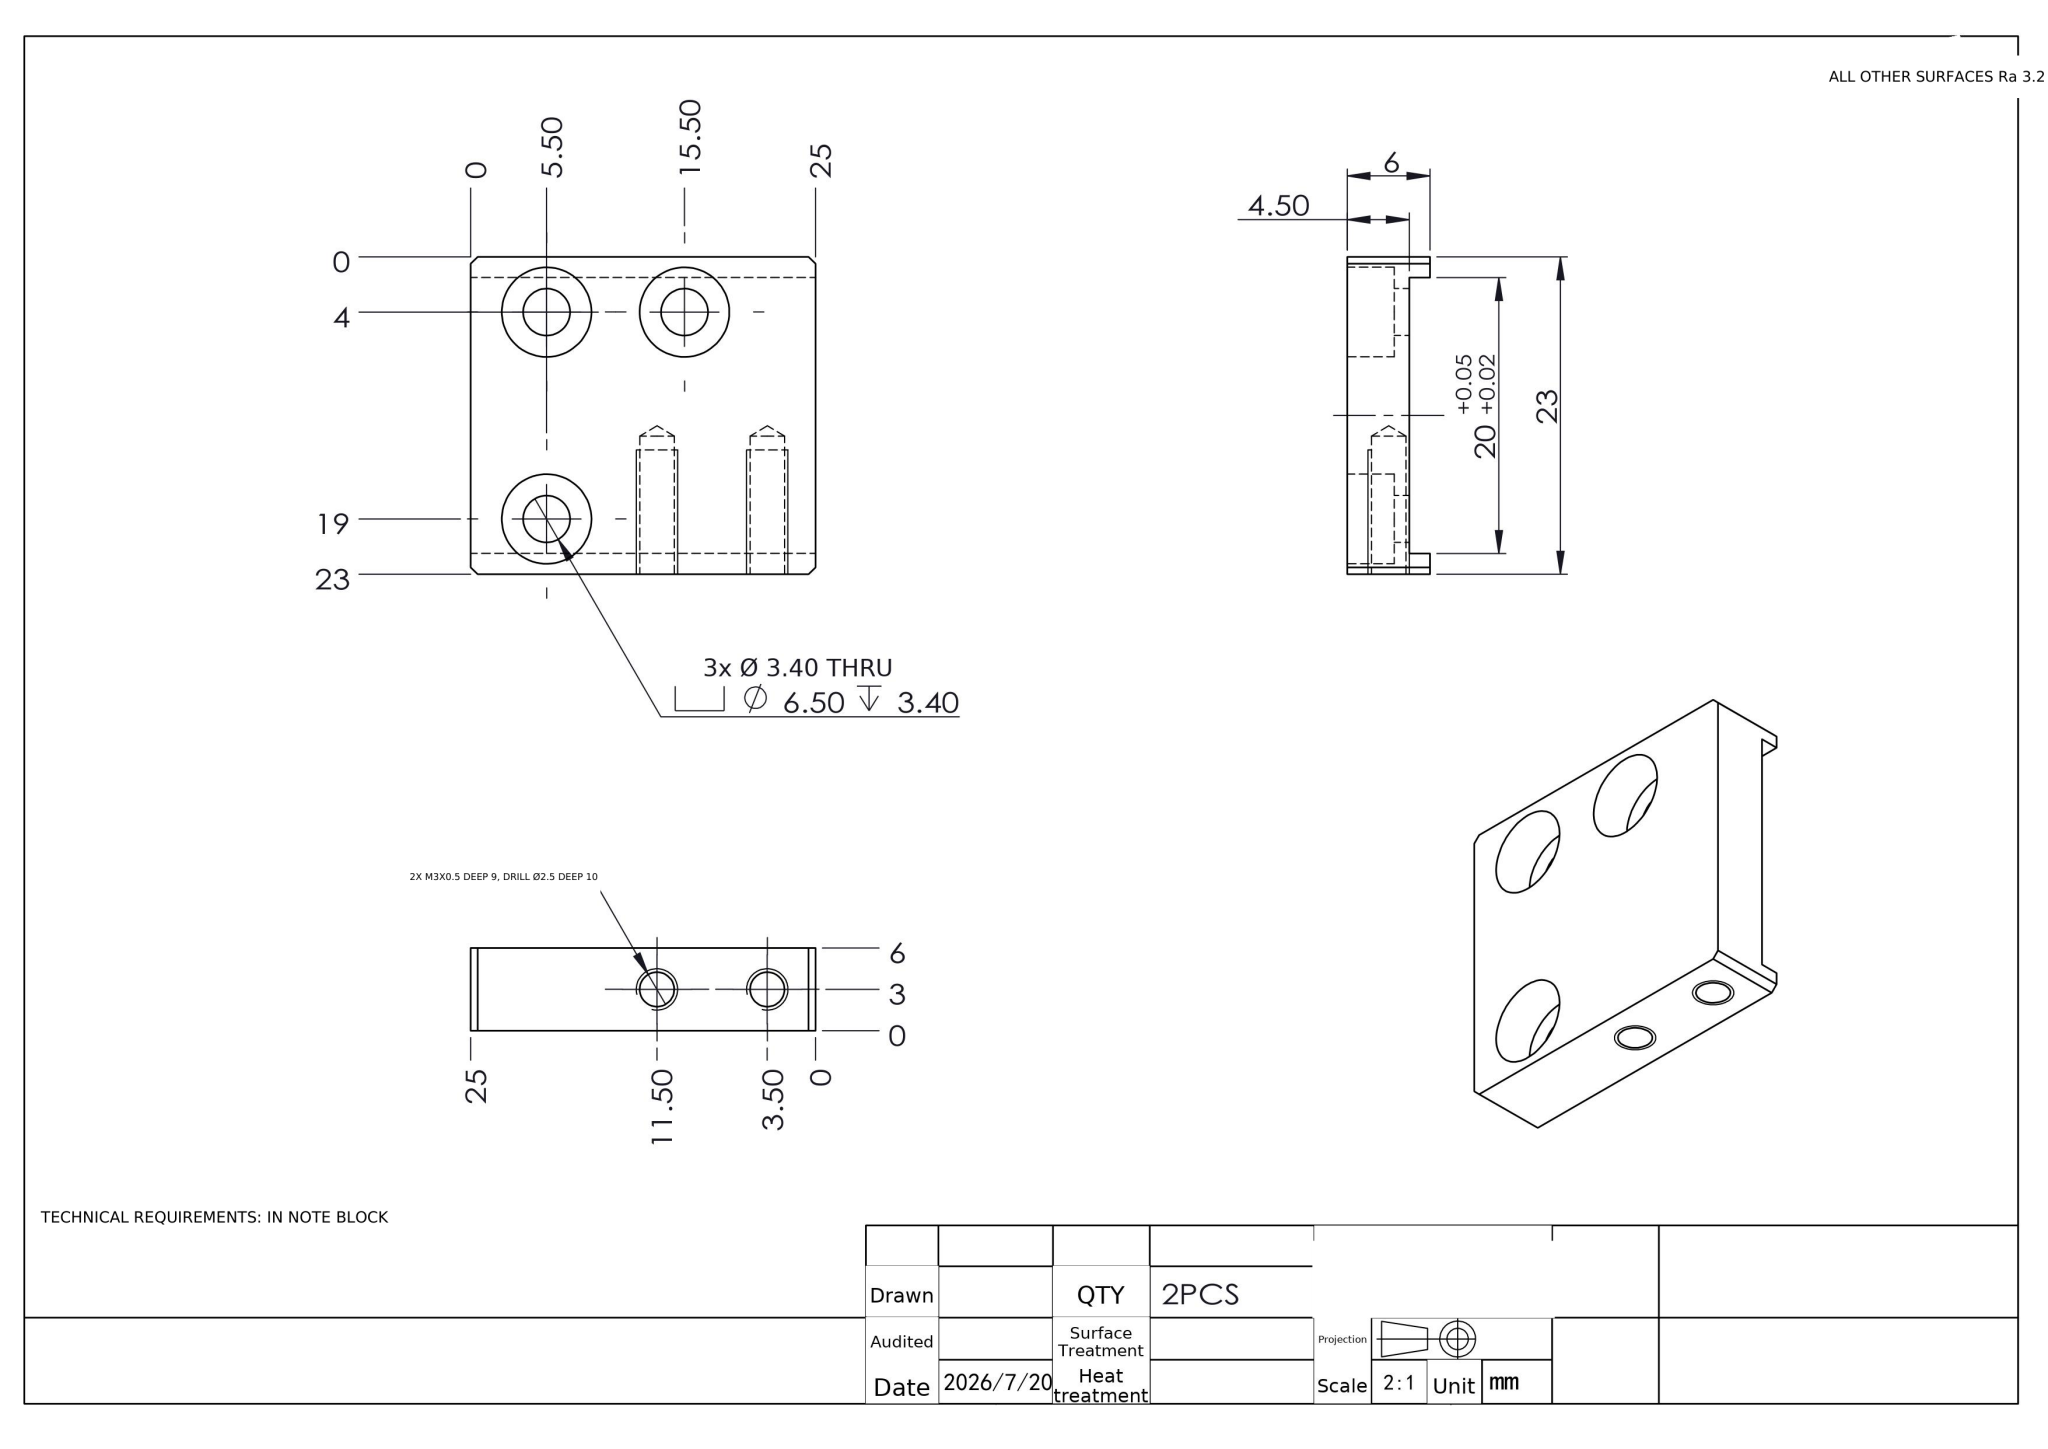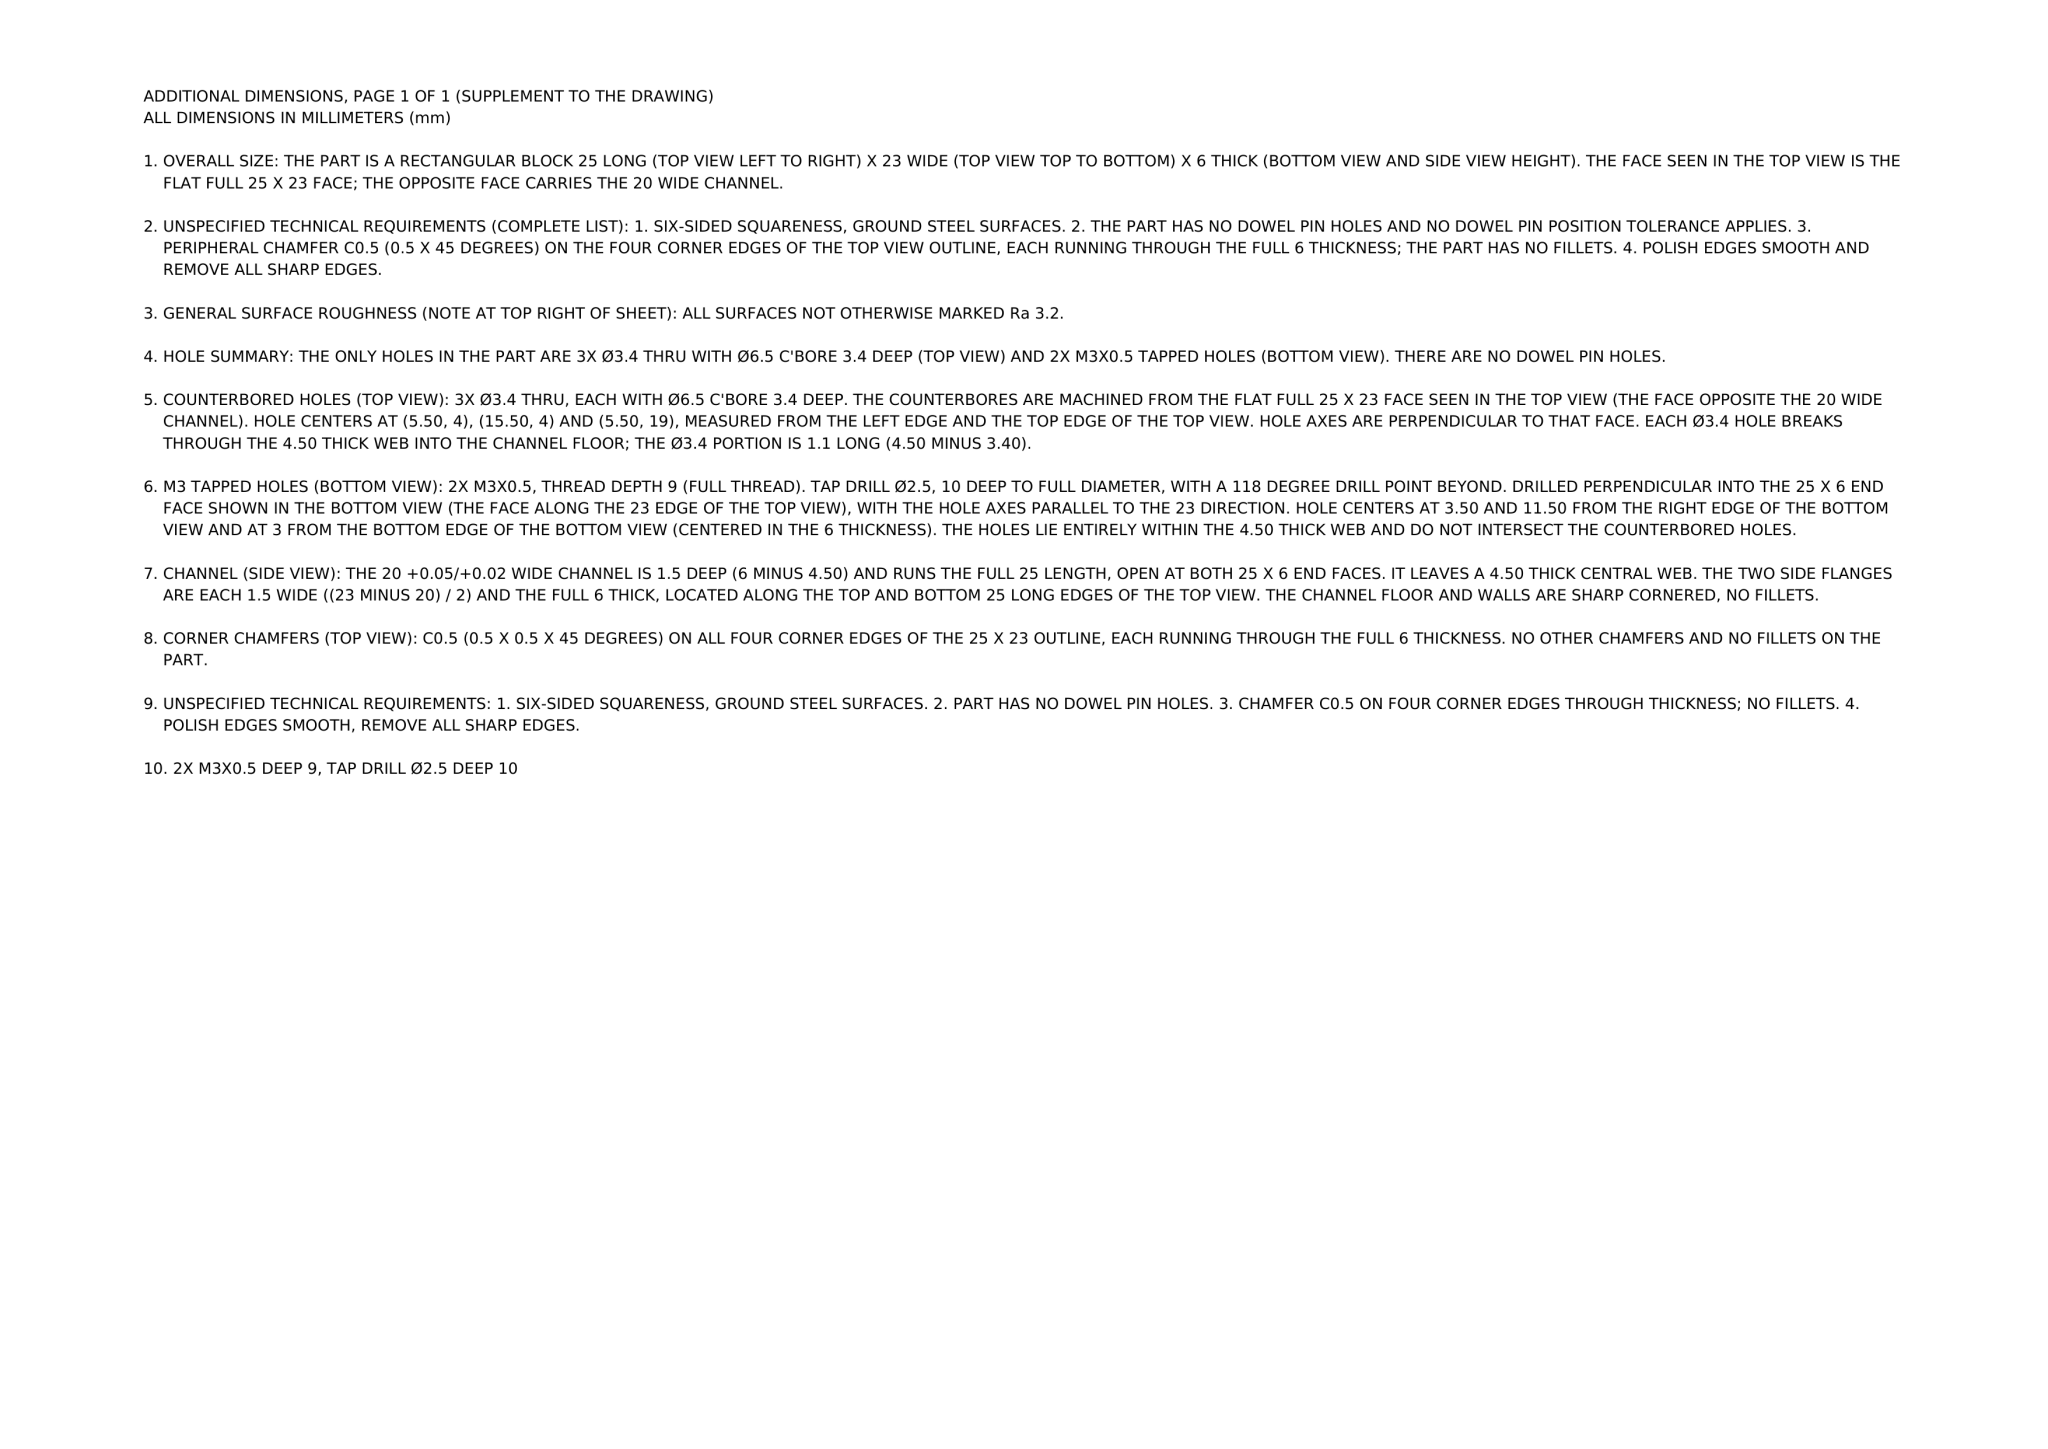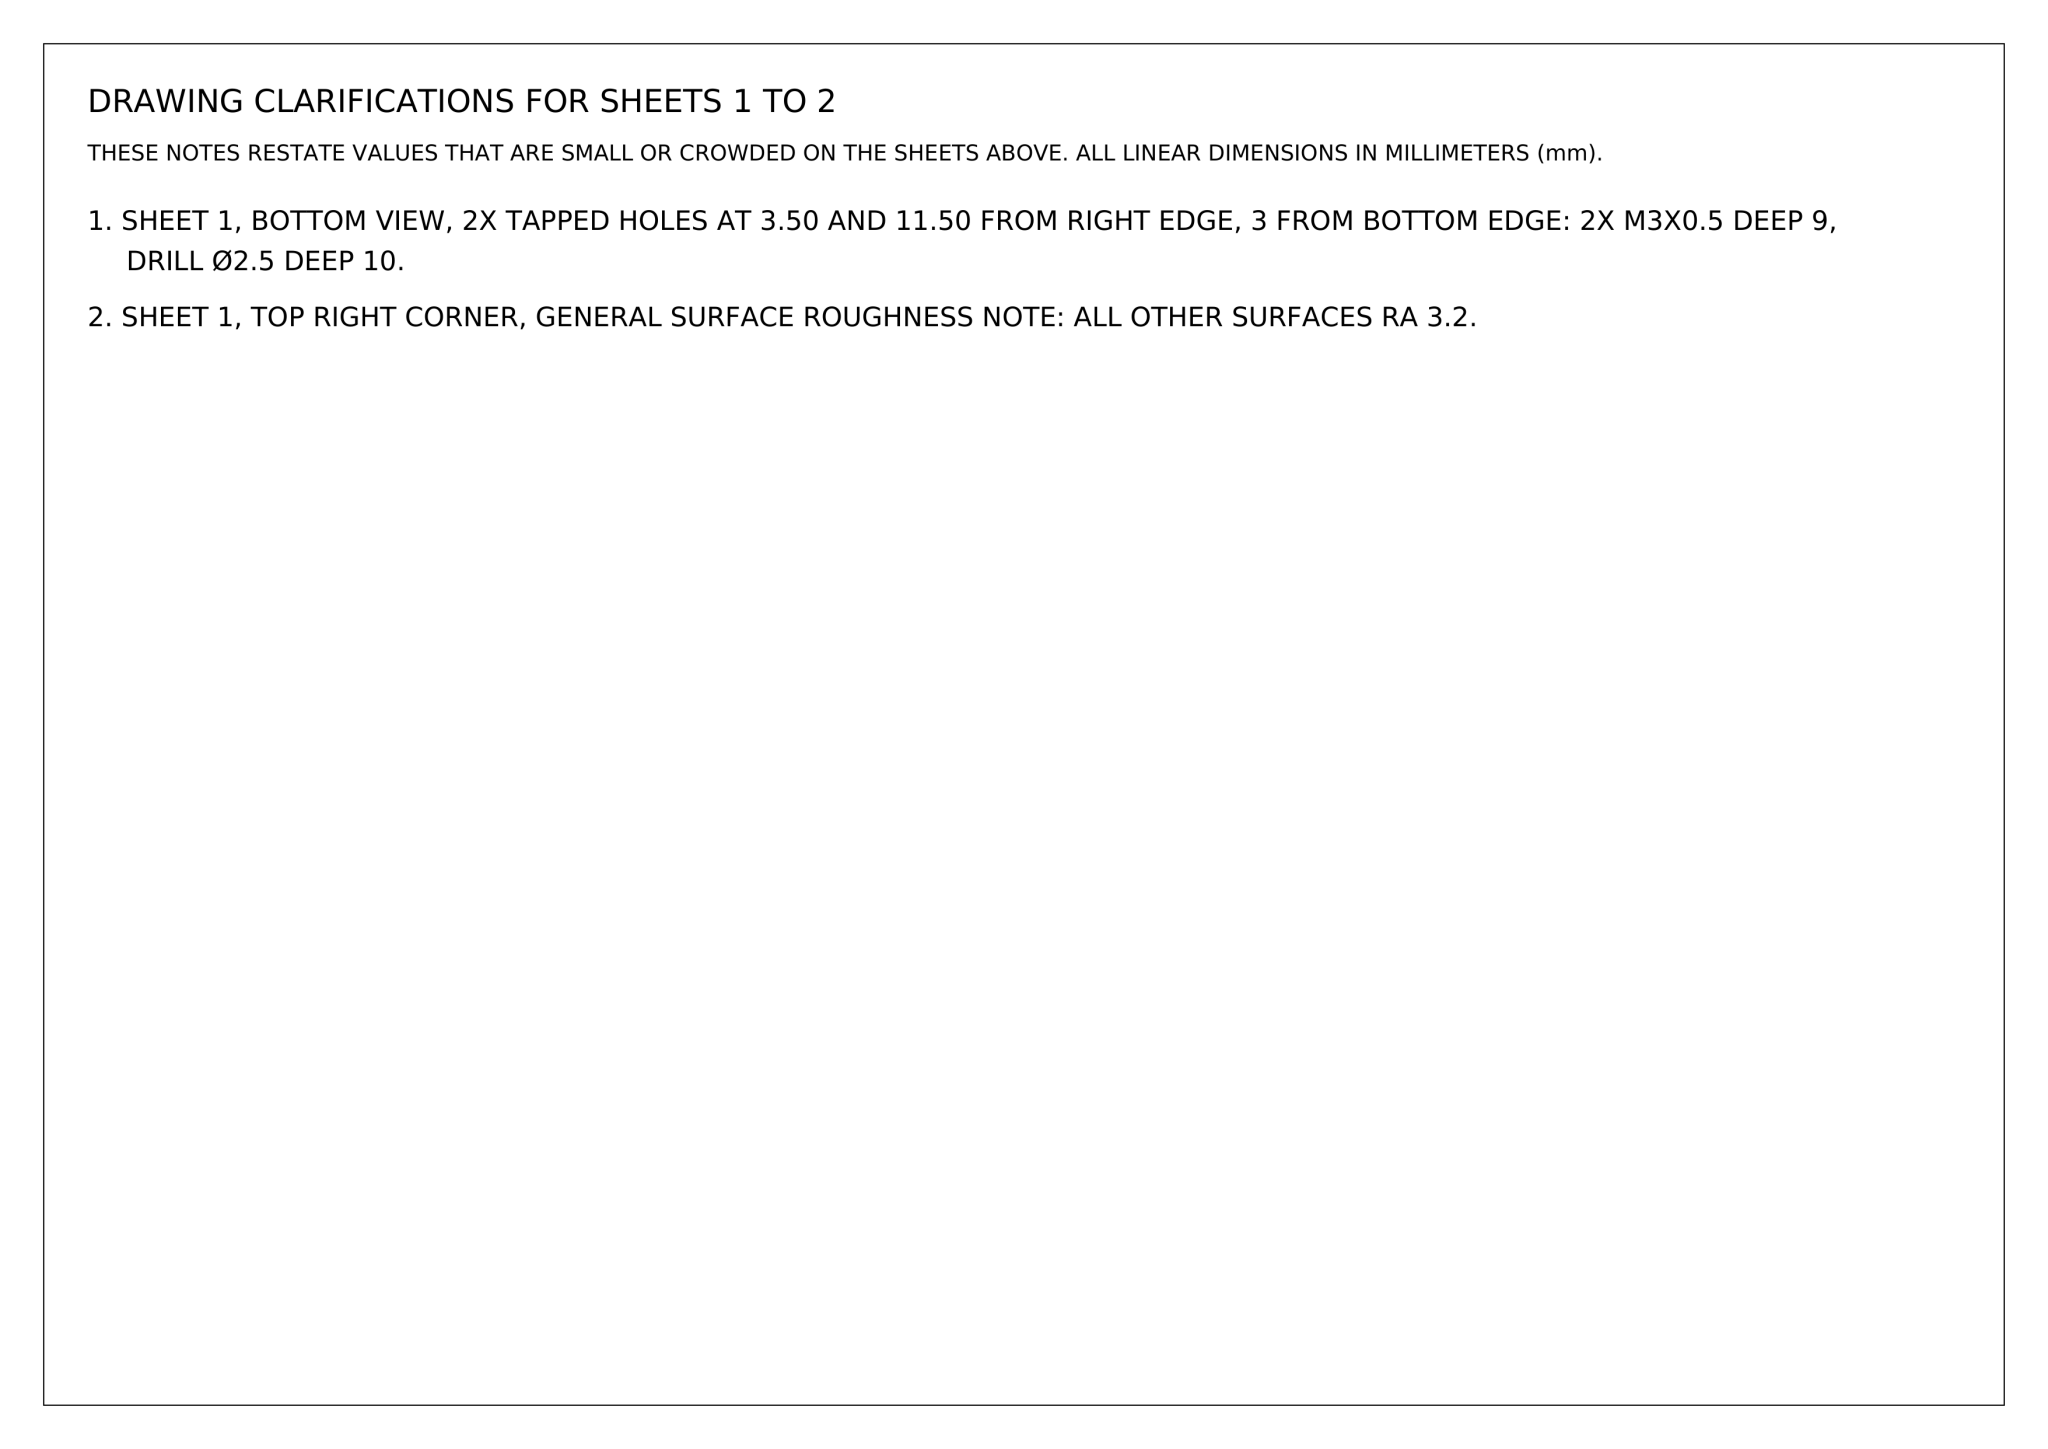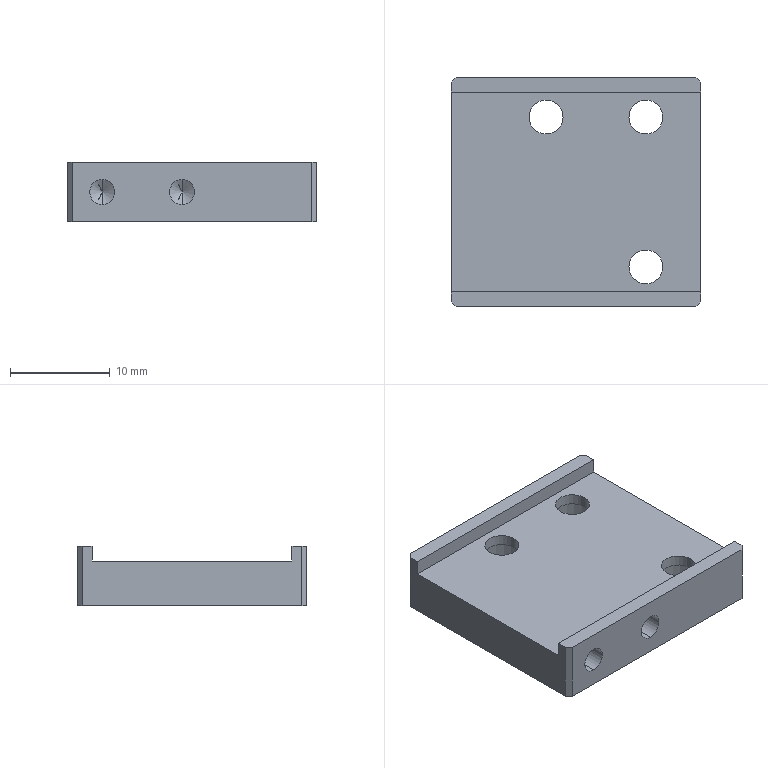Part | NX | mm | 1 solid | 37 faces | box 25 x 23 x 6 mm | volume 2228 mm3 | plane 17 | cylinder 16 | cone 4 | commonest cylinder face diameters 6.5 x6 3.4 x6 2.5 x4